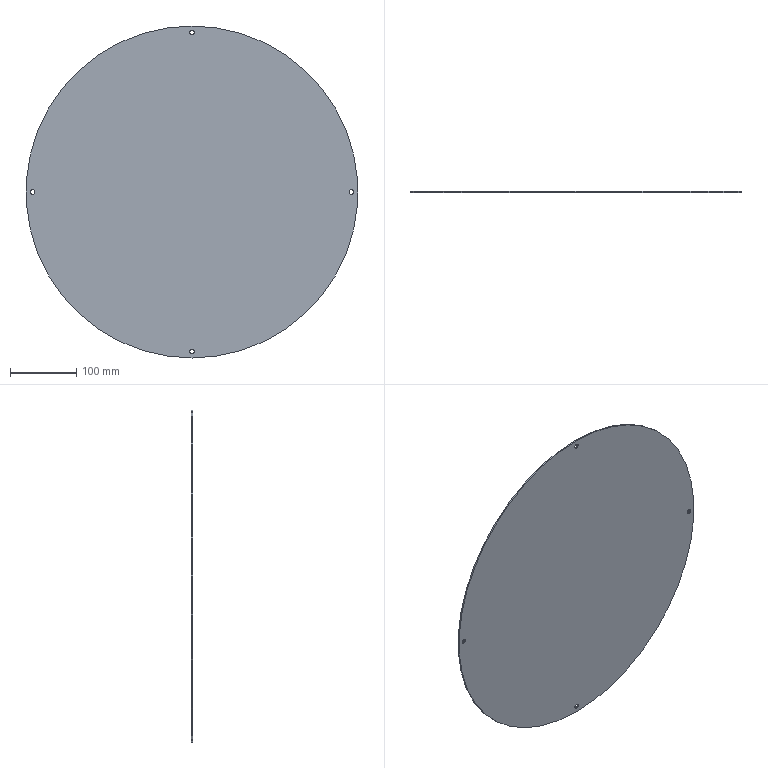Component | SolidWorks | CoverPlate-100_RoundPlate-1 | 1 solid | 12 faces | box 500 x 2 x 500 mm | volume 392391 mm3 | cylinder 10 | plane 2 | commonest cylinder face diameters 7 x8 500 x2 | material Plain Carbon Steel
STEP:
#1=CARTESIAN_POINT('',(-14.979,139.438,249.037));
#2=VERTEX_POINT('',#1);
#3=CARTESIAN_POINT('',(-14.979,139.438,249.313));
#4=VERTEX_POINT('',#3);
#5=CARTESIAN_POINT('',(-14.979,139.438,249.175));
#6=DIRECTION('',(0.,1.,0.));
#7=DIRECTION('',(0.,0.,-1.));
#8=AXIS2_PLACEMENT_3D('',#5,#6,#7);
#9=CIRCLE('',#8,0.1378);
#10=EDGE_CURVE('',#2,#4,#9,.T.);
#11=ORIENTED_EDGE('',*,*,#10,.F.);
#12=CARTESIAN_POINT('',(-14.979,139.517,249.037));
#13=VERTEX_POINT('',#12);
#14=CARTESIAN_POINT('',(-14.979,139.438,249.037));
#15=DIRECTION('',(0.,1.,0.));
#16=VECTOR('',#15,39.37);
#17=LINE('',#14,#16);
#18=EDGE_CURVE('',#2,#13,#17,.T.);
#19=ORIENTED_EDGE('',*,*,#18,.T.);
#20=CARTESIAN_POINT('',(-14.979,139.517,249.313));
#21=VERTEX_POINT('',#20);
#22=CARTESIAN_POINT('',(-14.979,139.517,249.175));
#23=DIRECTION('',(0.,1.,0.));
#24=DIRECTION('',(0.,0.,-1.));
#25=AXIS2_PLACEMENT_3D('',#22,#23,#24);
#26=CIRCLE('',#25,0.1378);
#27=EDGE_CURVE('',#13,#21,#26,.T.);
#28=ORIENTED_EDGE('',*,*,#27,.T.);
#29=CARTESIAN_POINT('',(-14.979,139.438,249.313));
#30=DIRECTION('',(0.,1.,0.));
#31=VECTOR('',#30,39.37);
#32=LINE('',#29,#31);
#33=EDGE_CURVE('',#4,#21,#32,.T.);
#34=ORIENTED_EDGE('',*,*,#33,.F.);
#35=EDGE_LOOP('',(#11,#19,#28,#34));
#36=FACE_OUTER_BOUND('',#35,.T.);
#37=CARTESIAN_POINT('',(-14.979,139.438,249.175));
#38=DIRECTION('',(0.,1.,0.));
#39=DIRECTION('',(0.,0.,1.));
#40=AXIS2_PLACEMENT_3D('',#37,#38,#39);
#41=CYLINDRICAL_SURFACE('',#40,0.1378);
#42=ADVANCED_FACE('',(#36),#41,.F.);
#43=CARTESIAN_POINT('',(-24.428,139.438,239.588));
#44=VERTEX_POINT('',#43);
#45=CARTESIAN_POINT('',(-24.428,139.438,239.864));
#46=VERTEX_POINT('',#45);
#47=CARTESIAN_POINT('',(-24.428,139.438,239.726));
#48=DIRECTION('',(0.,1.,0.));
#49=DIRECTION('',(0.,0.,-1.));
#50=AXIS2_PLACEMENT_3D('',#47,#48,#49);
#51=CIRCLE('',#50,0.1378);
#52=EDGE_CURVE('',#44,#46,#51,.T.);
#53=ORIENTED_EDGE('',*,*,#52,.F.);
#54=CARTESIAN_POINT('',(-24.428,139.517,239.588));
#55=VERTEX_POINT('',#54);
#56=CARTESIAN_POINT('',(-24.428,139.438,239.588));
#57=DIRECTION('',(0.,1.,0.));
#58=VECTOR('',#57,39.37);
#59=LINE('',#56,#58);
#60=EDGE_CURVE('',#44,#55,#59,.T.);
#61=ORIENTED_EDGE('',*,*,#60,.T.);
#62=CARTESIAN_POINT('',(-24.428,139.517,239.864));
#63=VERTEX_POINT('',#62);
#64=CARTESIAN_POINT('',(-24.428,139.517,239.726));
#65=DIRECTION('',(0.,1.,0.));
#66=DIRECTION('',(0.,0.,-1.));
#67=AXIS2_PLACEMENT_3D('',#64,#65,#66);
#68=CIRCLE('',#67,0.1378);
#69=EDGE_CURVE('',#55,#63,#68,.T.);
#70=ORIENTED_EDGE('',*,*,#69,.T.);
#71=CARTESIAN_POINT('',(-24.428,139.438,239.864));
#72=DIRECTION('',(0.,1.,0.));
#73=VECTOR('',#72,39.37);
#74=LINE('',#71,#73);
#75=EDGE_CURVE('',#46,#63,#74,.T.);
#76=ORIENTED_EDGE('',*,*,#75,.F.);
#77=EDGE_LOOP('',(#53,#61,#70,#76));
#78=FACE_OUTER_BOUND('',#77,.T.);
#79=CARTESIAN_POINT('',(-24.428,139.438,239.726));
#80=DIRECTION('',(0.,1.,0.));
#81=DIRECTION('',(0.,0.,1.));
#82=AXIS2_PLACEMENT_3D('',#79,#80,#81);
#83=CYLINDRICAL_SURFACE('',#82,0.1378);
#84=ADVANCED_FACE('',(#78),#83,.F.);
#85=CARTESIAN_POINT('',(-5.53,139.438,239.588));
#86=VERTEX_POINT('',#85);
#87=CARTESIAN_POINT('',(-5.53,139.438,239.864));
#88=VERTEX_POINT('',#87);
#89=CARTESIAN_POINT('',(-5.53,139.438,239.726));
#90=DIRECTION('',(0.,1.,0.));
#91=DIRECTION('',(0.,0.,1.));
#92=AXIS2_PLACEMENT_3D('',#89,#90,#91);
#93=CIRCLE('',#92,0.1378);
#94=EDGE_CURVE('',#86,#88,#93,.T.);
#95=ORIENTED_EDGE('',*,*,#94,.F.);
#96=CARTESIAN_POINT('',(-5.53,139.517,239.588));
#97=VERTEX_POINT('',#96);
#98=CARTESIAN_POINT('',(-5.53,139.438,239.588));
#99=DIRECTION('',(0.,1.,0.));
#100=VECTOR('',#99,39.37);
#101=LINE('',#98,#100);
#102=EDGE_CURVE('',#86,#97,#101,.T.);
#103=ORIENTED_EDGE('',*,*,#102,.T.);
#104=CARTESIAN_POINT('',(-5.53,139.517,239.864));
#105=VERTEX_POINT('',#104);
#106=CARTESIAN_POINT('',(-5.53,139.517,239.726));
#107=DIRECTION('',(0.,1.,0.));
#108=DIRECTION('',(0.,0.,1.));
#109=AXIS2_PLACEMENT_3D('',#106,#107,#108);
#110=CIRCLE('',#109,0.1378);
#111=EDGE_CURVE('',#97,#105,#110,.T.);
#112=ORIENTED_EDGE('',*,*,#111,.T.);
#113=CARTESIAN_POINT('',(-5.53,139.438,239.864));
#114=DIRECTION('',(0.,1.,0.));
#115=VECTOR('',#114,39.37);
#116=LINE('',#113,#115);
#117=EDGE_CURVE('',#88,#105,#116,.T.);
#118=ORIENTED_EDGE('',*,*,#117,.F.);
#119=EDGE_LOOP('',(#95,#103,#112,#118));
#120=FACE_OUTER_BOUND('',#119,.T.);
#121=CARTESIAN_POINT('',(-5.53,139.438,239.726));
#122=DIRECTION('',(0.,1.,0.));
#123=DIRECTION('',(0.,0.,1.));
#124=AXIS2_PLACEMENT_3D('',#121,#122,#123);
#125=CYLINDRICAL_SURFACE('',#124,0.1378);
#126=ADVANCED_FACE('',(#120),#125,.F.);
#127=CARTESIAN_POINT('',(-14.979,139.438,230.139));
#128=VERTEX_POINT('',#127);
#129=CARTESIAN_POINT('',(-14.979,139.438,230.415));
#130=VERTEX_POINT('',#129);
#131=CARTESIAN_POINT('',(-14.979,139.438,230.277));
#132=DIRECTION('',(0.,1.,0.));
#133=DIRECTION('',(0.,0.,1.));
#134=AXIS2_PLACEMENT_3D('',#131,#132,#133);
#135=CIRCLE('',#134,0.1378);
#136=EDGE_CURVE('',#128,#130,#135,.T.);
#137=ORIENTED_EDGE('',*,*,#136,.F.);
#138=CARTESIAN_POINT('',(-14.979,139.517,230.139));
#139=VERTEX_POINT('',#138);
#140=CARTESIAN_POINT('',(-14.979,139.438,230.139));
#141=DIRECTION('',(0.,1.,0.));
#142=VECTOR('',#141,39.37);
#143=LINE('',#140,#142);
#144=EDGE_CURVE('',#128,#139,#143,.T.);
#145=ORIENTED_EDGE('',*,*,#144,.T.);
#146=CARTESIAN_POINT('',(-14.979,139.517,230.415));
#147=VERTEX_POINT('',#146);
#148=CARTESIAN_POINT('',(-14.979,139.517,230.277));
#149=DIRECTION('',(0.,1.,0.));
#150=DIRECTION('',(0.,0.,1.));
#151=AXIS2_PLACEMENT_3D('',#148,#149,#150);
#152=CIRCLE('',#151,0.1378);
#153=EDGE_CURVE('',#139,#147,#152,.T.);
#154=ORIENTED_EDGE('',*,*,#153,.T.);
#155=CARTESIAN_POINT('',(-14.979,139.438,230.415));
#156=DIRECTION('',(0.,1.,0.));
#157=VECTOR('',#156,39.37);
#158=LINE('',#155,#157);
#159=EDGE_CURVE('',#130,#147,#158,.T.);
#160=ORIENTED_EDGE('',*,*,#159,.F.);
#161=EDGE_LOOP('',(#137,#145,#154,#160));
#162=FACE_OUTER_BOUND('',#161,.T.);
#163=CARTESIAN_POINT('',(-14.979,139.438,230.277));
#164=DIRECTION('',(0.,1.,0.));
#165=DIRECTION('',(0.,0.,1.));
#166=AXIS2_PLACEMENT_3D('',#163,#164,#165);
#167=CYLINDRICAL_SURFACE('',#166,0.1378);
#168=ADVANCED_FACE('',(#162),#167,.F.);
#169=CARTESIAN_POINT('',(-14.979,139.438,249.569));
#170=VERTEX_POINT('',#169);
#171=CARTESIAN_POINT('',(-14.979,139.438,229.884));
#172=VERTEX_POINT('',#171);
#173=CARTESIAN_POINT('',(-14.979,139.438,239.726));
#174=DIRECTION('',(0.,1.,0.));
#175=DIRECTION('',(0.,0.,1.));
#176=AXIS2_PLACEMENT_3D('',#173,#174,#175);
#177=CIRCLE('',#176,9.843);
#178=EDGE_CURVE('',#170,#172,#177,.T.);
#179=ORIENTED_EDGE('',*,*,#178,.T.);
#180=CARTESIAN_POINT('',(-14.979,139.517,229.884));
#181=VERTEX_POINT('',#180);
#182=CARTESIAN_POINT('',(-14.979,139.438,229.884));
#183=DIRECTION('',(0.,1.,0.));
#184=VECTOR('',#183,39.37);
#185=LINE('',#182,#184);
#186=EDGE_CURVE('',#172,#181,#185,.T.);
#187=ORIENTED_EDGE('',*,*,#186,.T.);
#188=CARTESIAN_POINT('',(-14.979,139.517,249.569));
#189=VERTEX_POINT('',#188);
#190=CARTESIAN_POINT('',(-14.979,139.517,239.726));
#191=DIRECTION('',(0.,1.,0.));
#192=DIRECTION('',(0.,0.,1.));
#193=AXIS2_PLACEMENT_3D('',#190,#191,#192);
#194=CIRCLE('',#193,9.843);
#195=EDGE_CURVE('',#189,#181,#194,.T.);
#196=ORIENTED_EDGE('',*,*,#195,.F.);
#197=CARTESIAN_POINT('',(-14.979,139.438,249.569));
#198=DIRECTION('',(0.,1.,0.));
#199=VECTOR('',#198,39.37);
#200=LINE('',#197,#199);
#201=EDGE_CURVE('',#170,#189,#200,.T.);
#202=ORIENTED_EDGE('',*,*,#201,.F.);
#203=EDGE_LOOP('',(#179,#187,#196,#202));
#204=FACE_OUTER_BOUND('',#203,.T.);
#205=CARTESIAN_POINT('',(-14.979,139.438,239.726));
#206=DIRECTION('',(0.,1.,0.));
#207=DIRECTION('',(0.,0.,1.));
#208=AXIS2_PLACEMENT_3D('',#205,#206,#207);
#209=CYLINDRICAL_SURFACE('',#208,9.843);
#210=ADVANCED_FACE('',(#204),#209,.T.);
#211=ORIENTED_EDGE('',*,*,#186,.F.);
#212=CARTESIAN_POINT('',(-14.979,139.438,239.726));
#213=DIRECTION('',(0.,1.,0.));
#214=DIRECTION('',(0.,0.,1.));
#215=AXIS2_PLACEMENT_3D('',#212,#213,#214);
#216=CIRCLE('',#215,9.843);
#217=EDGE_CURVE('',#172,#170,#216,.T.);
#218=ORIENTED_EDGE('',*,*,#217,.T.);
#219=ORIENTED_EDGE('',*,*,#201,.T.);
#220=CARTESIAN_POINT('',(-14.979,139.517,239.726));
#221=DIRECTION('',(0.,1.,0.));
#222=DIRECTION('',(0.,0.,1.));
#223=AXIS2_PLACEMENT_3D('',#220,#221,#222);
#224=CIRCLE('',#223,9.843);
#225=EDGE_CURVE('',#181,#189,#224,.T.);
#226=ORIENTED_EDGE('',*,*,#225,.F.);
#227=EDGE_LOOP('',(#211,#218,#219,#226));
#228=FACE_OUTER_BOUND('',#227,.T.);
#229=CARTESIAN_POINT('',(-14.979,139.438,239.726));
#230=DIRECTION('',(0.,1.,0.));
#231=DIRECTION('',(0.,0.,1.));
#232=AXIS2_PLACEMENT_3D('',#229,#230,#231);
#233=CYLINDRICAL_SURFACE('',#232,9.843);
#234=ADVANCED_FACE('',(#228),#233,.T.);
#235=CARTESIAN_POINT('',(-14.979,139.438,249.175));
#236=DIRECTION('',(0.,1.,0.));
#237=DIRECTION('',(0.,0.,-1.));
#238=AXIS2_PLACEMENT_3D('',#235,#236,#237);
#239=CIRCLE('',#238,0.1378);
#240=EDGE_CURVE('',#4,#2,#239,.T.);
#241=ORIENTED_EDGE('',*,*,#240,.T.);
#242=ORIENTED_EDGE('',*,*,#10,.T.);
#243=EDGE_LOOP('',(#241,#242));
#244=FACE_BOUND('',#243,.T.);
#245=CARTESIAN_POINT('',(-24.428,139.438,239.726));
#246=DIRECTION('',(0.,1.,0.));
#247=DIRECTION('',(0.,0.,-1.));
#248=AXIS2_PLACEMENT_3D('',#245,#246,#247);
#249=CIRCLE('',#248,0.1378);
#250=EDGE_CURVE('',#46,#44,#249,.T.);
#251=ORIENTED_EDGE('',*,*,#250,.T.);
#252=ORIENTED_EDGE('',*,*,#52,.T.);
#253=EDGE_LOOP('',(#251,#252));
#254=FACE_BOUND('',#253,.T.);
#255=CARTESIAN_POINT('',(-5.53,139.438,239.726));
#256=DIRECTION('',(0.,1.,0.));
#257=DIRECTION('',(0.,0.,1.));
#258=AXIS2_PLACEMENT_3D('',#255,#256,#257);
#259=CIRCLE('',#258,0.1378);
#260=EDGE_CURVE('',#88,#86,#259,.T.);
#261=ORIENTED_EDGE('',*,*,#260,.T.);
#262=ORIENTED_EDGE('',*,*,#94,.T.);
#263=EDGE_LOOP('',(#261,#262));
#264=FACE_BOUND('',#263,.T.);
#265=CARTESIAN_POINT('',(-14.979,139.438,230.277));
#266=DIRECTION('',(0.,1.,0.));
#267=DIRECTION('',(0.,0.,1.));
#268=AXIS2_PLACEMENT_3D('',#265,#266,#267);
#269=CIRCLE('',#268,0.1378);
#270=EDGE_CURVE('',#130,#128,#269,.T.);
#271=ORIENTED_EDGE('',*,*,#270,.T.);
#272=ORIENTED_EDGE('',*,*,#136,.T.);
#273=EDGE_LOOP('',(#271,#272));
#274=FACE_BOUND('',#273,.T.);
#275=ORIENTED_EDGE('',*,*,#178,.F.);
#276=ORIENTED_EDGE('',*,*,#217,.F.);
#277=EDGE_LOOP('',(#275,#276));
#278=FACE_OUTER_BOUND('',#277,.T.);
#279=CARTESIAN_POINT('',(-14.979,139.438,239.726));
#280=DIRECTION('',(0.,1.,0.));
#281=DIRECTION('',(0.,0.,1.));
#282=AXIS2_PLACEMENT_3D('',#279,#280,#281);
#283=PLANE('',#282);
#284=ADVANCED_FACE('',(#244,#254,#264,#274,#278),#283,.F.);
#285=CARTESIAN_POINT('',(-14.979,139.517,249.175));
#286=DIRECTION('',(0.,1.,0.));
#287=DIRECTION('',(0.,0.,-1.));
#288=AXIS2_PLACEMENT_3D('',#285,#286,#287);
#289=CIRCLE('',#288,0.1378);
#290=EDGE_CURVE('',#21,#13,#289,.T.);
#291=ORIENTED_EDGE('',*,*,#290,.F.);
#292=ORIENTED_EDGE('',*,*,#27,.F.);
#293=EDGE_LOOP('',(#291,#292));
#294=FACE_BOUND('',#293,.T.);
#295=CARTESIAN_POINT('',(-24.428,139.517,239.726));
#296=DIRECTION('',(0.,1.,0.));
#297=DIRECTION('',(0.,0.,-1.));
#298=AXIS2_PLACEMENT_3D('',#295,#296,#297);
#299=CIRCLE('',#298,0.1378);
#300=EDGE_CURVE('',#63,#55,#299,.T.);
#301=ORIENTED_EDGE('',*,*,#300,.F.);
#302=ORIENTED_EDGE('',*,*,#69,.F.);
#303=EDGE_LOOP('',(#301,#302));
#304=FACE_BOUND('',#303,.T.);
#305=CARTESIAN_POINT('',(-5.53,139.517,239.726));
#306=DIRECTION('',(0.,1.,0.));
#307=DIRECTION('',(0.,0.,1.));
#308=AXIS2_PLACEMENT_3D('',#305,#306,#307);
#309=CIRCLE('',#308,0.1378);
#310=EDGE_CURVE('',#105,#97,#309,.T.);
#311=ORIENTED_EDGE('',*,*,#310,.F.);
#312=ORIENTED_EDGE('',*,*,#111,.F.);
#313=EDGE_LOOP('',(#311,#312));
#314=FACE_BOUND('',#313,.T.);
#315=CARTESIAN_POINT('',(-14.979,139.517,230.277));
#316=DIRECTION('',(0.,1.,0.));
#317=DIRECTION('',(0.,0.,1.));
#318=AXIS2_PLACEMENT_3D('',#315,#316,#317);
#319=CIRCLE('',#318,0.1378);
#320=EDGE_CURVE('',#147,#139,#319,.T.);
#321=ORIENTED_EDGE('',*,*,#320,.F.);
#322=ORIENTED_EDGE('',*,*,#153,.F.);
#323=EDGE_LOOP('',(#321,#322));
#324=FACE_BOUND('',#323,.T.);
#325=ORIENTED_EDGE('',*,*,#195,.T.);
#326=ORIENTED_EDGE('',*,*,#225,.T.);
#327=EDGE_LOOP('',(#325,#326));
#328=FACE_OUTER_BOUND('',#327,.T.);
#329=CARTESIAN_POINT('',(-14.979,139.517,239.726));
#330=DIRECTION('',(0.,1.,0.));
#331=DIRECTION('',(0.,0.,1.));
#332=AXIS2_PLACEMENT_3D('',#329,#330,#331);
#333=PLANE('',#332);
#334=ADVANCED_FACE('',(#294,#304,#314,#324,#328),#333,.T.);
#335=ORIENTED_EDGE('',*,*,#144,.F.);
#336=ORIENTED_EDGE('',*,*,#270,.F.);
#337=ORIENTED_EDGE('',*,*,#159,.T.);
#338=ORIENTED_EDGE('',*,*,#320,.T.);
#339=EDGE_LOOP('',(#335,#336,#337,#338));
#340=FACE_OUTER_BOUND('',#339,.T.);
#341=CARTESIAN_POINT('',(-14.979,139.438,230.277));
#342=DIRECTION('',(0.,1.,0.));
#343=DIRECTION('',(0.,0.,1.));
#344=AXIS2_PLACEMENT_3D('',#341,#342,#343);
#345=CYLINDRICAL_SURFACE('',#344,0.1378);
#346=ADVANCED_FACE('',(#340),#345,.F.);
#347=ORIENTED_EDGE('',*,*,#102,.F.);
#348=ORIENTED_EDGE('',*,*,#260,.F.);
#349=ORIENTED_EDGE('',*,*,#117,.T.);
#350=ORIENTED_EDGE('',*,*,#310,.T.);
#351=EDGE_LOOP('',(#347,#348,#349,#350));
#352=FACE_OUTER_BOUND('',#351,.T.);
#353=CARTESIAN_POINT('',(-5.53,139.438,239.726));
#354=DIRECTION('',(0.,1.,0.));
#355=DIRECTION('',(0.,0.,1.));
#356=AXIS2_PLACEMENT_3D('',#353,#354,#355);
#357=CYLINDRICAL_SURFACE('',#356,0.1378);
#358=ADVANCED_FACE('',(#352),#357,.F.);
#359=ORIENTED_EDGE('',*,*,#60,.F.);
#360=ORIENTED_EDGE('',*,*,#250,.F.);
#361=ORIENTED_EDGE('',*,*,#75,.T.);
#362=ORIENTED_EDGE('',*,*,#300,.T.);
#363=EDGE_LOOP('',(#359,#360,#361,#362));
#364=FACE_OUTER_BOUND('',#363,.T.);
#365=CARTESIAN_POINT('',(-24.428,139.438,239.726));
#366=DIRECTION('',(0.,1.,0.));
#367=DIRECTION('',(0.,0.,1.));
#368=AXIS2_PLACEMENT_3D('',#365,#366,#367);
#369=CYLINDRICAL_SURFACE('',#368,0.1378);
#370=ADVANCED_FACE('',(#364),#369,.F.);
#371=ORIENTED_EDGE('',*,*,#18,.F.);
#372=ORIENTED_EDGE('',*,*,#240,.F.);
#373=ORIENTED_EDGE('',*,*,#33,.T.);
#374=ORIENTED_EDGE('',*,*,#290,.T.);
#375=EDGE_LOOP('',(#371,#372,#373,#374));
#376=FACE_OUTER_BOUND('',#375,.T.);
#377=CARTESIAN_POINT('',(-14.979,139.438,249.175));
#378=DIRECTION('',(0.,1.,0.));
#379=DIRECTION('',(0.,0.,1.));
#380=AXIS2_PLACEMENT_3D('',#377,#378,#379);
#381=CYLINDRICAL_SURFACE('',#380,0.1378);
#382=ADVANCED_FACE('',(#376),#381,.F.);
#383=CLOSED_SHELL('',(#42,#84,#126,#168,#210,#234,#284,#334,#346,#358,#370,#382));
#384=MANIFOLD_SOLID_BREP('',#383);
#385=CARTESIAN_POINT('',(0.,0.,0.));
#386=DIRECTION('',(0.,0.,1.));
#387=DIRECTION('',(1.,0.,0.));
#388=AXIS2_PLACEMENT_3D('',#385,#386,#387);
#389=(LENGTH_UNIT()NAMED_UNIT(*)SI_UNIT($,.METRE.));
#390=LENGTH_MEASURE_WITH_UNIT(LENGTH_MEASURE(0.0254),#389);
#391=DIMENSIONAL_EXPONENTS(1.,0.,0.,0.,0.,0.,0.);
#392=(CONVERSION_BASED_UNIT('',#390)LENGTH_UNIT()NAMED_UNIT(#391));
#393=UNCERTAINTY_MEASURE_WITH_UNIT(LENGTH_MEASURE(0.00001),#392,'','');
#394=(NAMED_UNIT(*)PLANE_ANGLE_UNIT()SI_UNIT($,.RADIAN.));
#395=(NAMED_UNIT(*)SI_UNIT($,.STERADIAN.)SOLID_ANGLE_UNIT());
#396=(GEOMETRIC_REPRESENTATION_CONTEXT(3)GLOBAL_UNCERTAINTY_ASSIGNED_CONTEXT((#393))GLOBAL_UNIT_ASSIGNED_CONTEXT((#392,#394,#395))REPRESENTATION_CONTEXT('',''));
#397=ADVANCED_BREP_SHAPE_REPRESENTATION('',(#384,#388),#396);
#398=COLOUR_RGB('',0.7922,0.8196,0.9333);
#399=FILL_AREA_STYLE_COLOUR('',#398);
#400=FILL_AREA_STYLE('',(#399));
#401=SURFACE_STYLE_FILL_AREA(#400);
#402=SURFACE_SIDE_STYLE('',(#401));
#403=SURFACE_STYLE_USAGE(.BOTH.,#402);
#404=PRESENTATION_STYLE_ASSIGNMENT((#403));
#405=STYLED_ITEM('',(#404),#384);
#406=PRESENTATION_LAYER_ASSIGNMENT('','',(#405));
#407=(LENGTH_UNIT()NAMED_UNIT(*)SI_UNIT($,.METRE.));
#408=LENGTH_MEASURE_WITH_UNIT(LENGTH_MEASURE(0.0254),#407);
#409=DIMENSIONAL_EXPONENTS(1.,0.,0.,0.,0.,0.,0.);
#410=(CONVERSION_BASED_UNIT('',#408)LENGTH_UNIT()NAMED_UNIT(#409));
#411=UNCERTAINTY_MEASURE_WITH_UNIT(LENGTH_MEASURE(0.00001),#410,'','');
#412=(NAMED_UNIT(*)PLANE_ANGLE_UNIT()SI_UNIT($,.RADIAN.));
#413=(NAMED_UNIT(*)SI_UNIT($,.STERADIAN.)SOLID_ANGLE_UNIT());
#414=(GEOMETRIC_REPRESENTATION_CONTEXT(3)GLOBAL_UNCERTAINTY_ASSIGNED_CONTEXT((#411))GLOBAL_UNIT_ASSIGNED_CONTEXT((#410,#412,#413))REPRESENTATION_CONTEXT('',''));
#415=MECHANICAL_DESIGN_GEOMETRIC_PRESENTATION_REPRESENTATION('',(#405),#414);